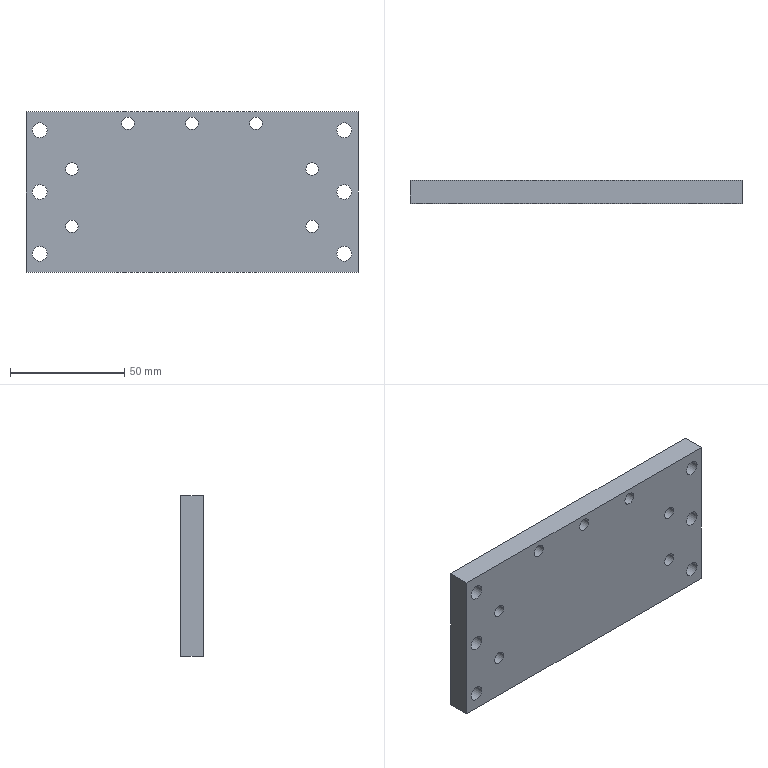Component | SolidWorks | LD101-02--Q1043-Q1-2-1 | 1 solid | 53 faces | box 145 x 10 x 70 mm | volume 96256 mm3 | cylinder 40 | plane 13 | commonest cylinder face diameters 9 x14 5.5 x14 6.5 x12 | material AL6061
build123d program:
from build123d import *

# Parameters (mm, degrees)
SKETCH1_W                                          = 145
SKETCH1_H                                          = 70
BOSS_EXTRUDE1_DEPTH                                = 5
HOLE_SIZE_FOR_HEX_SOCKET_HEAD_CAP_SCRE_D           = 5.5
HOLE_SIZE_FOR_HEX_SOCKET_HEAD_CAP_SCRE_CBORE_D     = 9
HOLE_SIZE_FOR_HEX_SOCKET_HEAD_CAP_SCRE_CBORE_DEPTH = 5.7
F_6_5_6_5_DIAMETER_HOLE1_D                         = 6.5


with BuildPart() as part:
    # Sketch1 → Boss-Extrude1 (new, symmetric)
    with BuildSketch(Plane.XY):
        Rectangle(SKETCH1_W, SKETCH1_H)
    extrude(amount=BOSS_EXTRUDE1_DEPTH, both=True)

    # Hole Size _for_ Hex Socket Head Cap Scre (through all)
    with Locations(Plane.XY.offset(5)):
        with Locations((-28, -30), (0, -30), (28, -30), (-52.5, 15), (52.5, 15), (-52.5, -10), (52.5, -10)):
            CounterBoreHole(HOLE_SIZE_FOR_HEX_SOCKET_HEAD_CAP_SCRE_D / 2, HOLE_SIZE_FOR_HEX_SOCKET_HEAD_CAP_SCRE_CBORE_D / 2, HOLE_SIZE_FOR_HEX_SOCKET_HEAD_CAP_SCRE_CBORE_DEPTH)

    # 6.5 _6.5_ Diameter Hole1 (through all)
    with Locations(Plane(origin=(0, 0, -5), x_dir=(-1, 0, 0), z_dir=(0, 0, -1))):
        with Locations((-66.5, 27), (-66.5, 0), (-66.5, -27), (66.5, 27), (66.5, 0), (66.5, -27)):
            Hole(F_6_5_6_5_DIAMETER_HOLE1_D / 2)


solid = part.part

# Placed as in the assembly
solid = solid.moved(Location((229.211, -256.897, 258.257), (-90, 0, 0)))